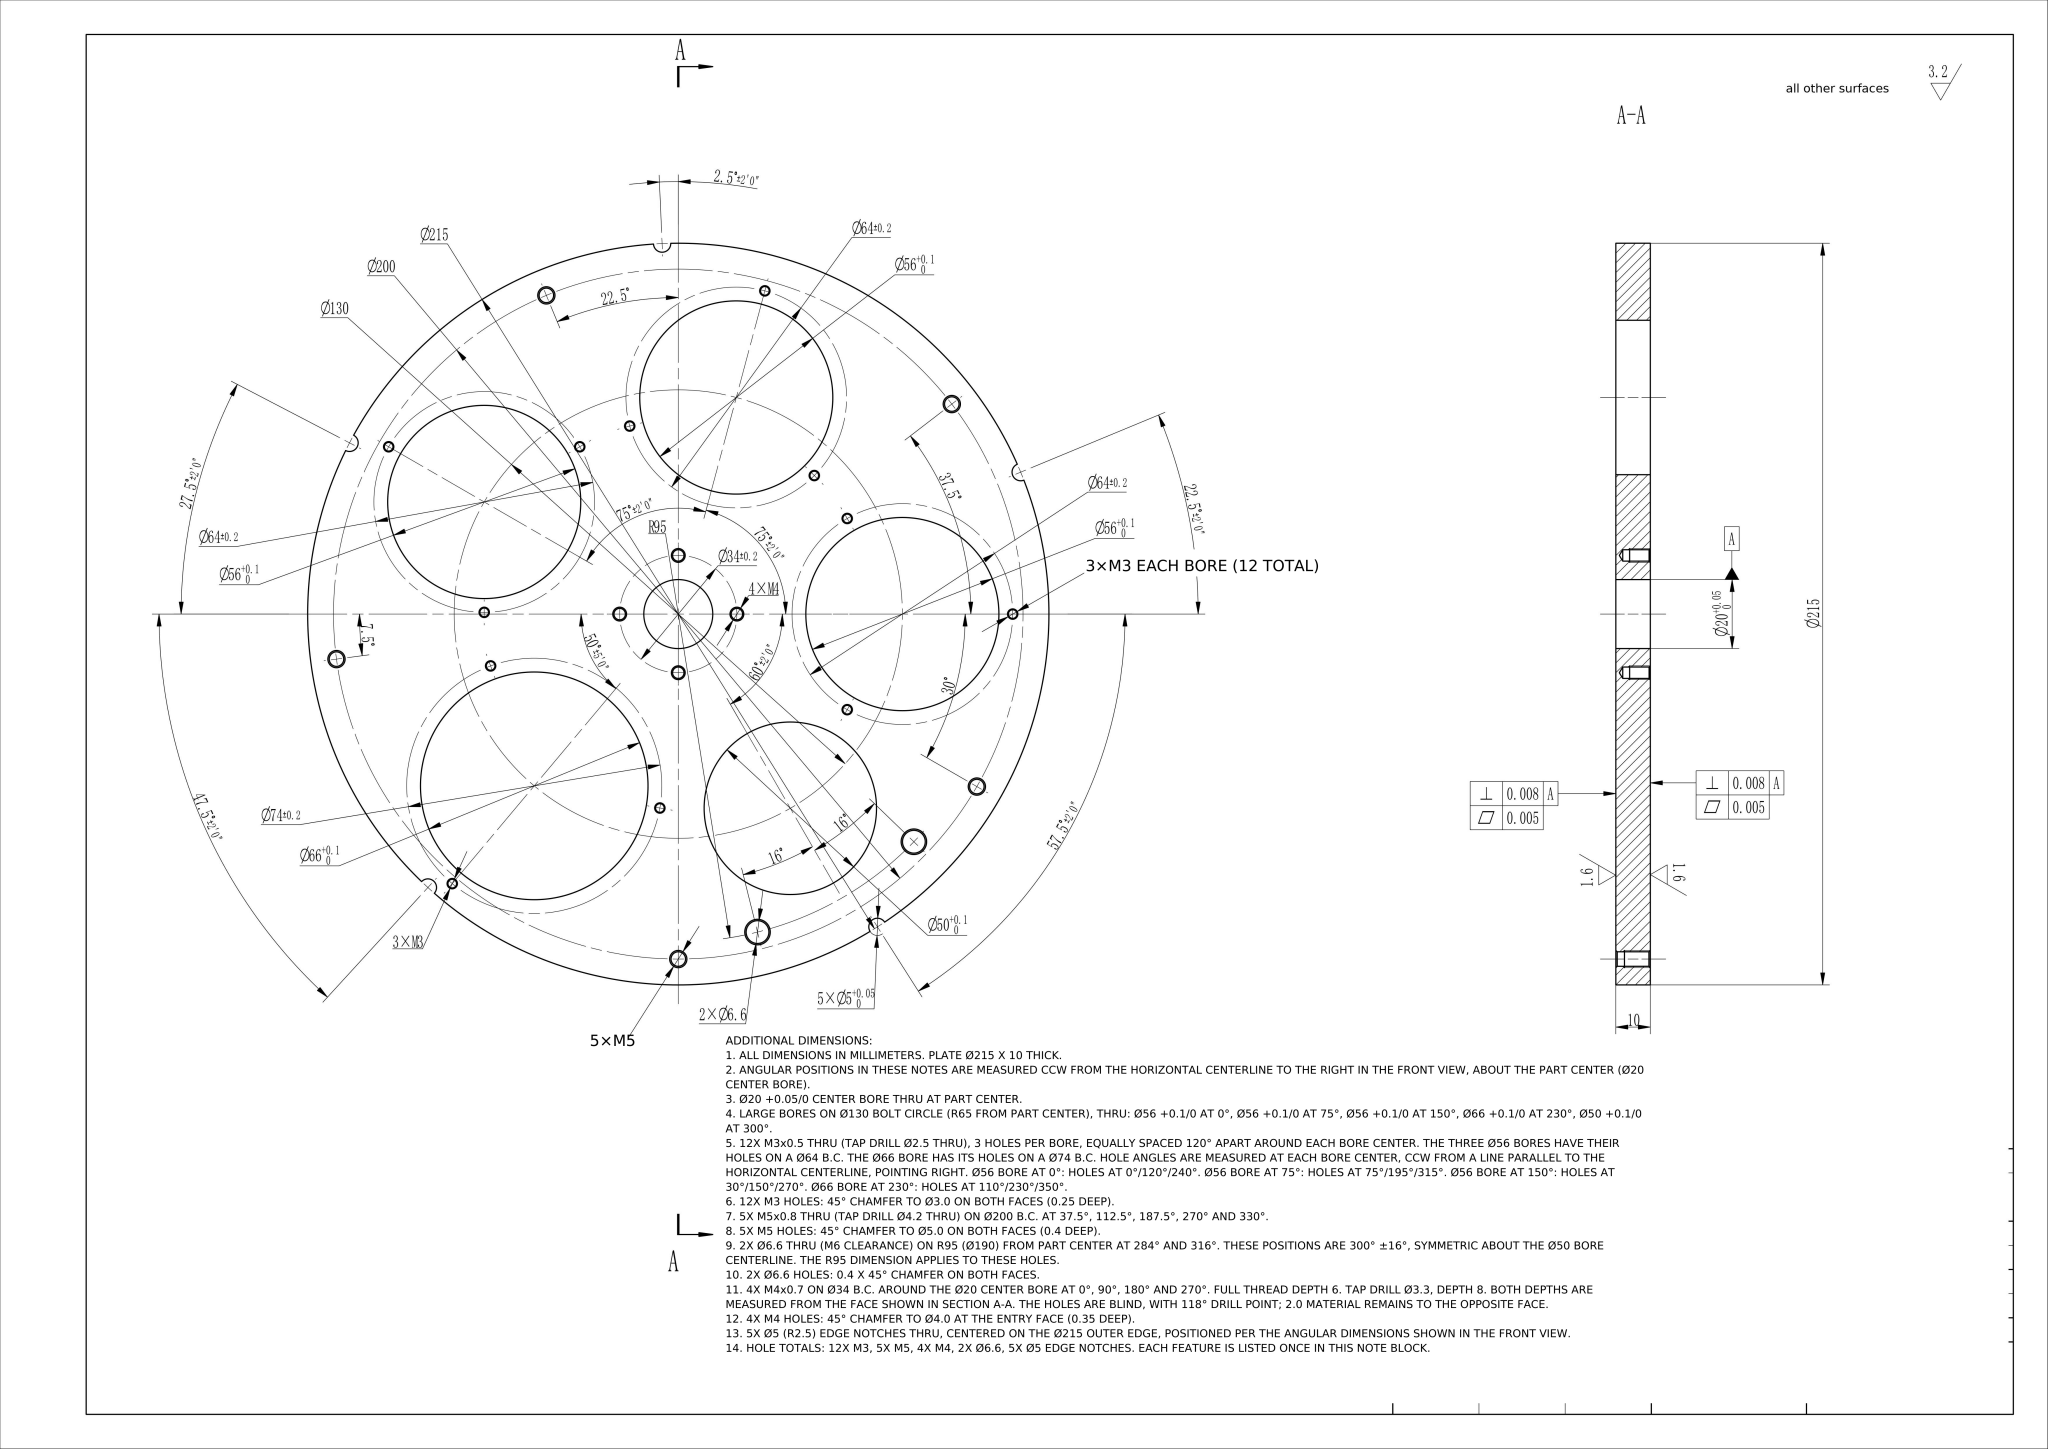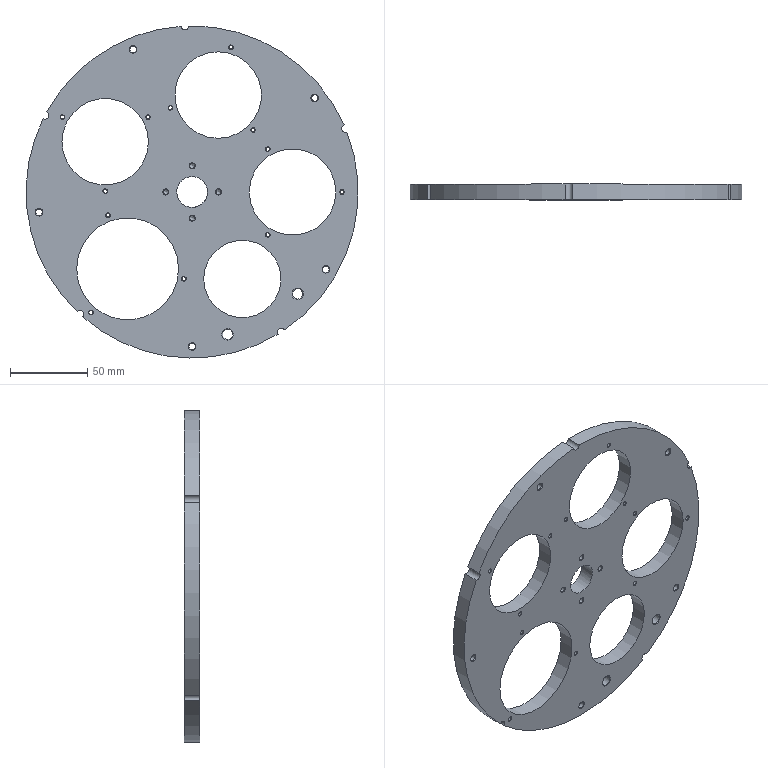Part | NX | mm | 1 solid | 87 faces | box 215 x 10 x 215 mm | volume 229405 mm3 | cone 46 | cylinder 39 | plane 2 | commonest cylinder face diameters 2.5 x12 215 x5 4.2 x5 5 x5 3.3 x4 56 x3 6.6 x2 66 x1